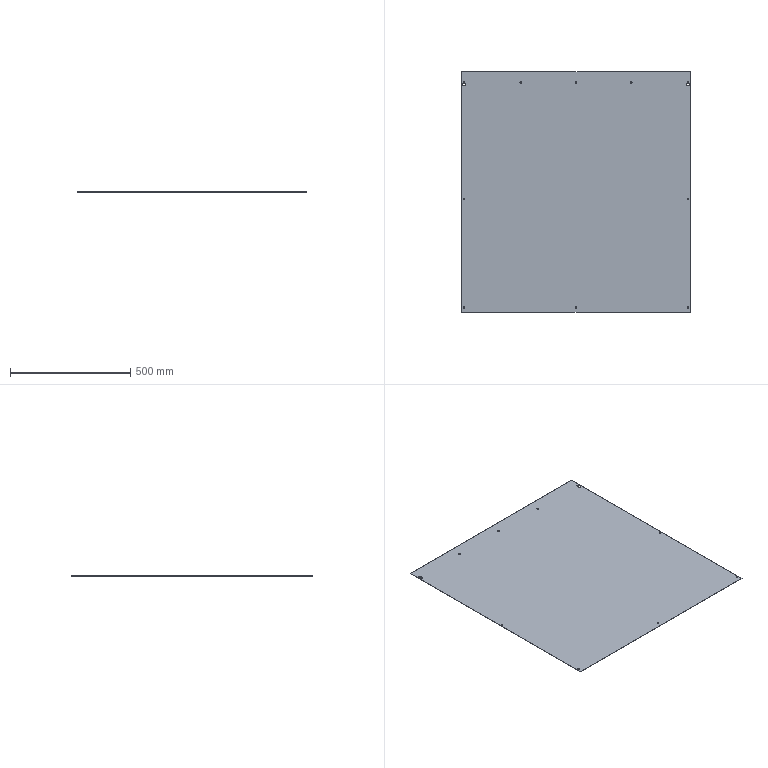Component | SolidWorks | SYM0671-81-106-2 | 1 solid | 34 faces | volume 1139383 mm3 | cylinder 24 | plane 10 | commonest cylinder face diameters 6 x18 12 x6 | material Plain Carbon Steel